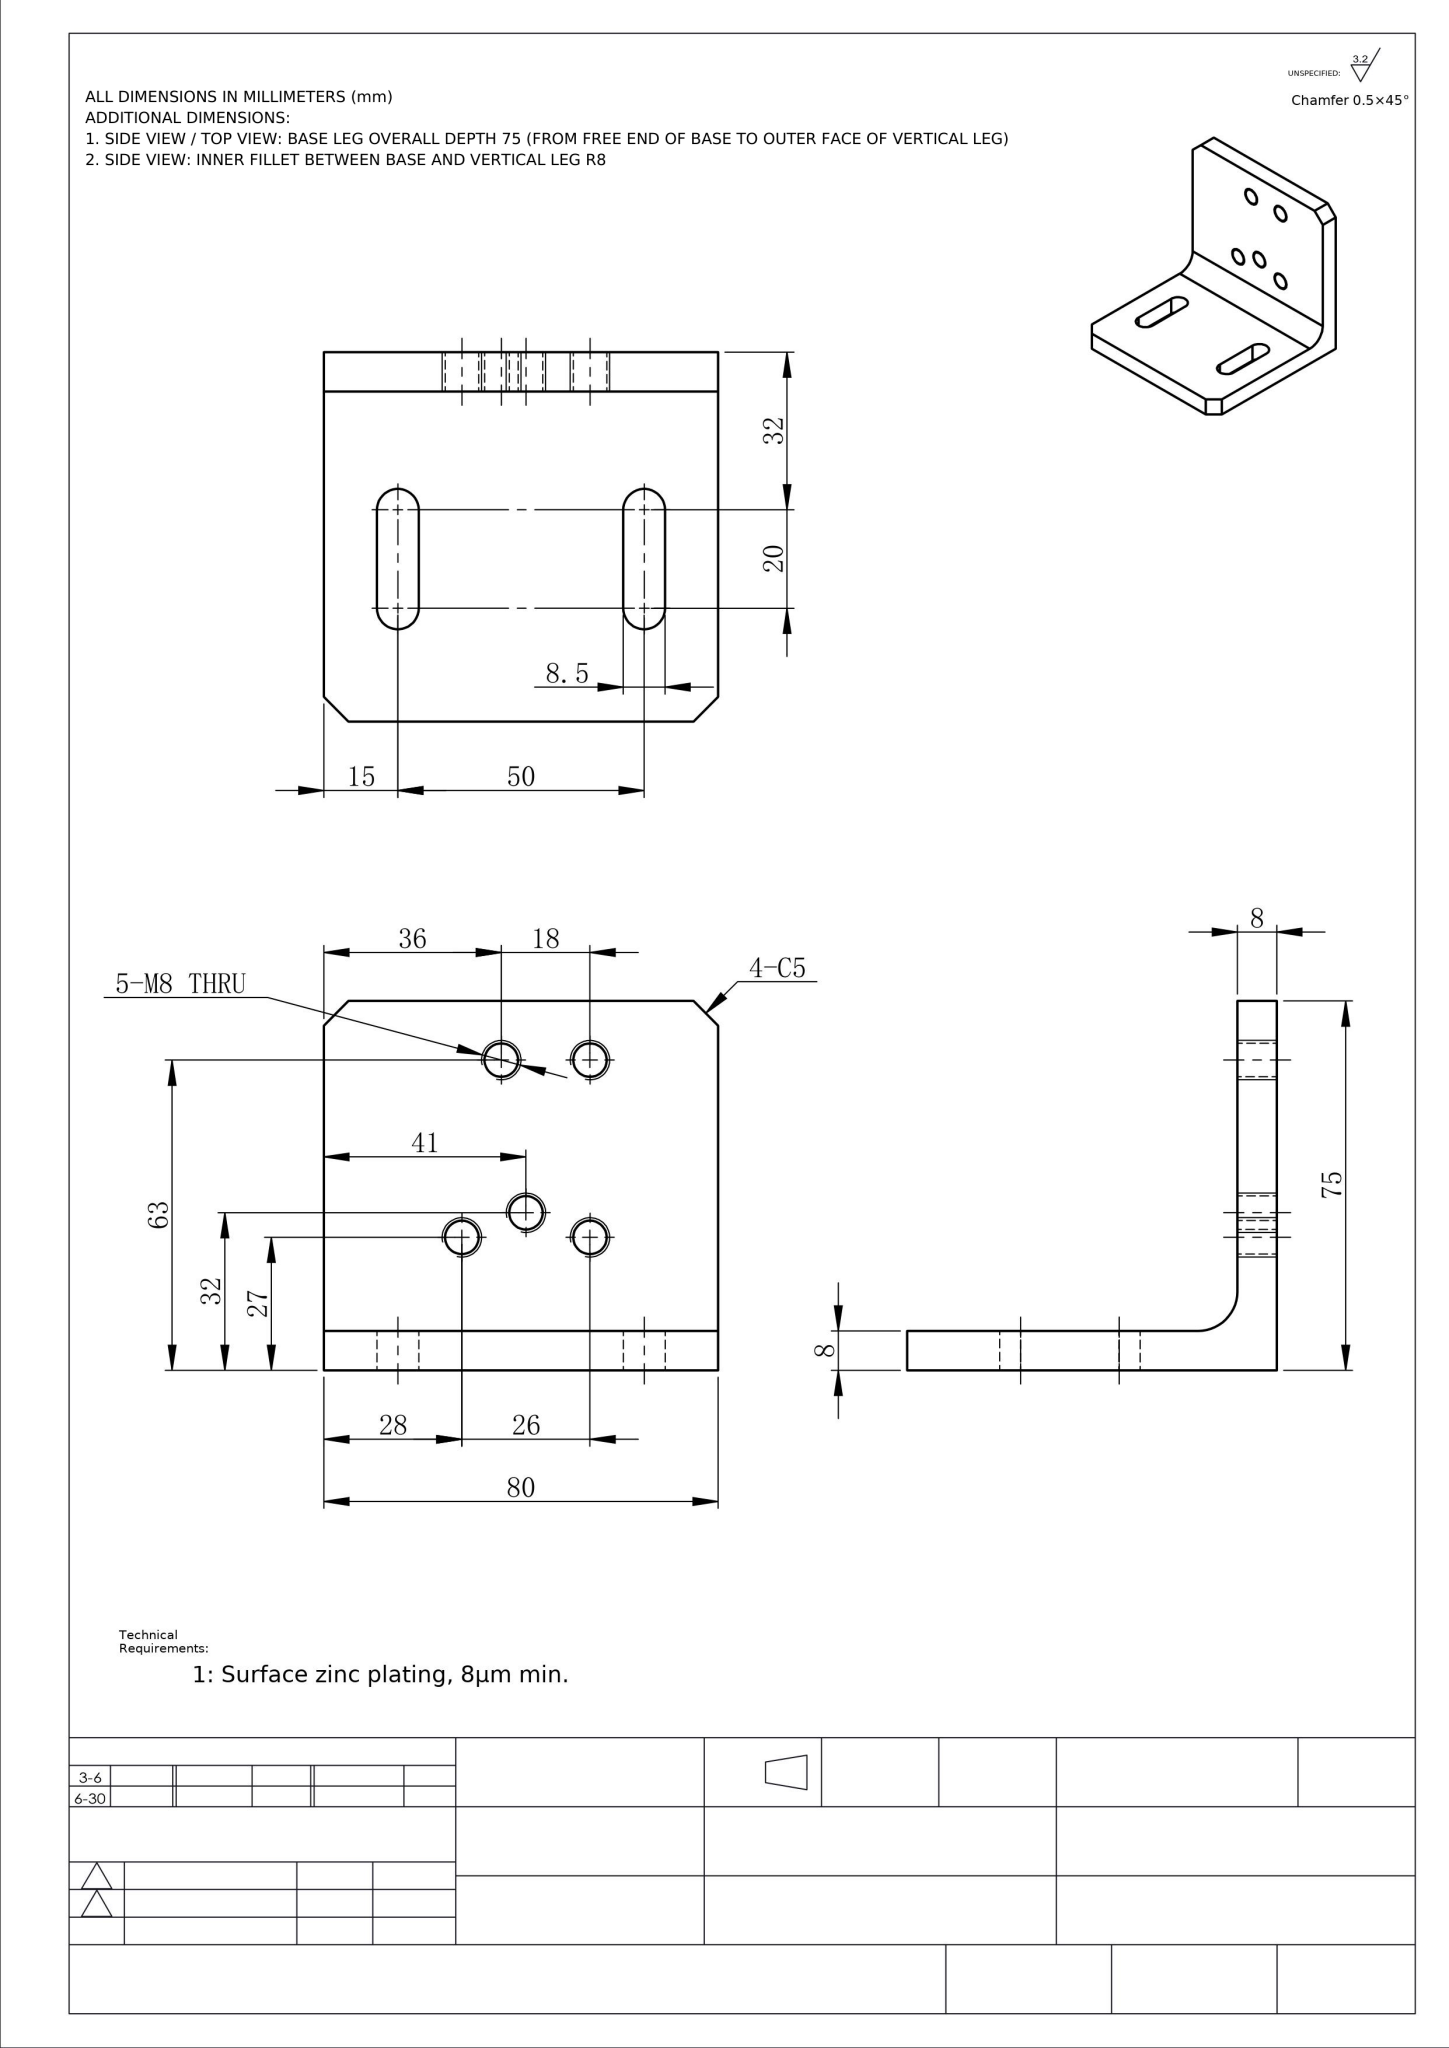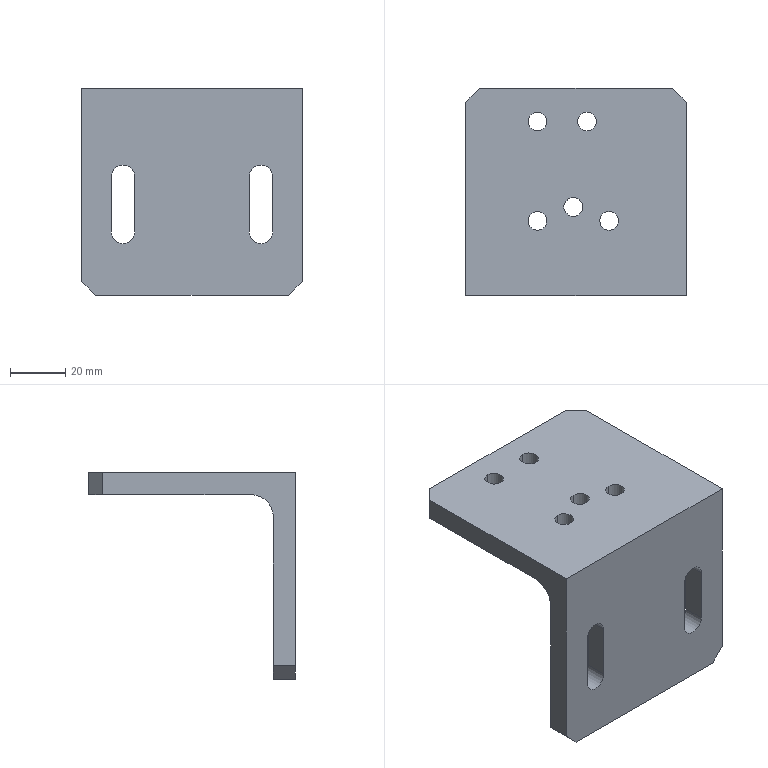Part | NX | mm | 1 solid | 33 faces | box 80 x 75 x 75 mm | volume 86498 mm3 | cylinder 17 | plane 16 | commonest cylinder face diameters 6.8 x10 8.5 x6 16 x1